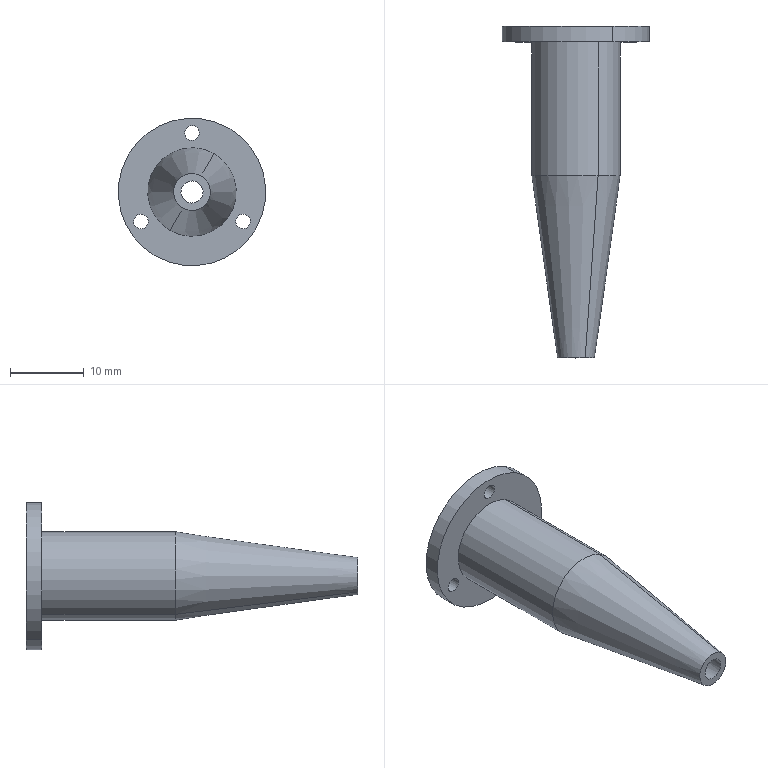Component | SolidWorks | Nozzle2-1 | 1 solid | 21 faces | box 20 x 45 x 20 mm | volume 1658 mm3 | cylinder 12 | cone 6 | plane 3 | commonest cylinder face diameters 2 x6 10 x2 20 x2 12 x2
build123d program:
from build123d import *

# Parameters (mm, degrees)
CUT_EXTRUDE1_REACH = 49.17
SKETCH2_R          = 1


with BuildPart() as part:
    # Sketch1 → Revolve1 (revolve)
    with BuildSketch(Plane.XY, mode=Mode.PRIVATE) as revolve1_sk:
        Polygon((-17.802, 0), (27.198, 0), (27.198, 2.5), (2.473, 6), (-15.659, 6), (-15.659, 10), (-17.802, 10), align=None)
    revolve(revolve1_sk.sketch.rotate(Axis((-17.802, 0, 0), (1, 0, 0)), 90), axis=Axis((-17.802, 0, 0), (1, 0, 0)))

    # Sketch2 → Cut-Extrude1 (cut, up to next)
    with BuildSketch(Plane.ZY.offset(17.802), mode=Mode.PRIVATE) as cut_extrude1_sk1:
        with Locations((0, 8)):
            Circle(SKETCH2_R)
    cut_extrude1_tool1 = extrude(cut_extrude1_sk1.sketch, amount=-CUT_EXTRUDE1_REACH, mode=Mode.PRIVATE) & part.part
    # Sketch2 → Cut-Extrude1 (cut, up to next)
    with BuildSketch(Plane.ZY.offset(17.802), mode=Mode.PRIVATE) as cut_extrude1_sk2:
        with Locations((6.928, -4)):
            Circle(SKETCH2_R)
    cut_extrude1_tool2 = extrude(cut_extrude1_sk2.sketch, amount=-CUT_EXTRUDE1_REACH, mode=Mode.PRIVATE) & part.part
    # Sketch2 → Cut-Extrude1 (cut, up to next)
    with BuildSketch(Plane.ZY.offset(17.802), mode=Mode.PRIVATE) as cut_extrude1_sk3:
        with Locations((-6.928, -4)):
            Circle(SKETCH2_R)
    cut_extrude1_tool3 = extrude(cut_extrude1_sk3.sketch, amount=-CUT_EXTRUDE1_REACH, mode=Mode.PRIVATE) & part.part
    add(cut_extrude1_tool1.solids().sort_by_distance((-17.802, 8, 0))[0], mode=Mode.SUBTRACT)
    add(cut_extrude1_tool2.solids().sort_by_distance((-17.802, -4, 6.928))[0], mode=Mode.SUBTRACT)
    add(cut_extrude1_tool3.solids().sort_by_distance((-17.802, -4, -6.928))[0], mode=Mode.SUBTRACT)

    # Sketch5 → Cut-Revolve1 (revolve, cut)
    with BuildSketch(Plane(origin=(0, 0, 0), x_dir=(1, 0, 0), z_dir=(0, 1, 0)), mode=Mode.PRIVATE) as cut_revolve1_sk:
        Polygon((-17.802, 0), (2.473, 0), (27.198, 0), (27.198, 1.5), (2.473, 5), (-15.659, 5), (-17.802, 6), align=None)
    revolve(cut_revolve1_sk.sketch.rotate(Axis((-17.802, 0, 0), (1, 0, 0)), 180), axis=Axis((-17.802, 0, 0), (1, 0, 0)), mode=Mode.SUBTRACT)


solid = part.part

# Placed as in the assembly
solid = solid.moved(Location((-5.981, -125.796, 160), (90, -90, 0)))
STEP:
#1=COLOUR_RGB('',0.7922,0.8196,0.9333);
#2=FILL_AREA_STYLE_COLOUR('',#1);
#3=FILL_AREA_STYLE('',(#2));
#4=SURFACE_STYLE_FILL_AREA(#3);
#5=SURFACE_SIDE_STYLE('',(#4));
#6=SURFACE_STYLE_USAGE(.BOTH.,#5);
#7=PRESENTATION_STYLE_ASSIGNMENT((#6));
#8=CARTESIAN_POINT('',(-0.3339,-4.336,6.129));
#9=VERTEX_POINT('',#8);
#10=CARTESIAN_POINT('',(-0.137,-4.336,6.47));
#11=VERTEX_POINT('',#10);
#12=CARTESIAN_POINT('',(-0.2355,-4.336,6.299));
#13=DIRECTION('',(-0.,1.,0.));
#14=DIRECTION('',(0.5,0.,0.866));
#15=AXIS2_PLACEMENT_3D('',#12,#13,#14);
#16=CIRCLE('',#15,0.1969);
#17=EDGE_CURVE('',#9,#11,#16,.T.);
#18=ORIENTED_EDGE('',*,*,#17,.F.);
#19=CARTESIAN_POINT('',(-0.3536,-4.252,6.095));
#20=VERTEX_POINT('',#19);
#21=CARTESIAN_POINT('',(-0.3339,-4.336,6.129));
#22=DIRECTION('',(-0.2114,0.9062,-0.3662));
#23=VECTOR('',#22,39.37);
#24=LINE('',#21,#23);
#25=EDGE_CURVE('',#9,#20,#24,.T.);
#26=ORIENTED_EDGE('',*,*,#25,.T.);
#27=CARTESIAN_POINT('',(-0.1174,-4.252,6.504));
#28=VERTEX_POINT('',#27);
#29=CARTESIAN_POINT('',(-0.2355,-4.252,6.299));
#30=DIRECTION('',(-0.,1.,0.));
#31=DIRECTION('',(0.5,0.,0.866));
#32=AXIS2_PLACEMENT_3D('',#29,#30,#31);
#33=CIRCLE('',#32,0.2362);
#34=EDGE_CURVE('',#20,#28,#33,.T.);
#35=ORIENTED_EDGE('',*,*,#34,.T.);
#36=CARTESIAN_POINT('',(-0.137,-4.336,6.47));
#37=DIRECTION('',(0.2114,0.9062,0.3662));
#38=VECTOR('',#37,39.37);
#39=LINE('',#36,#38);
#40=EDGE_CURVE('',#11,#28,#39,.T.);
#41=ORIENTED_EDGE('',*,*,#40,.F.);
#42=EDGE_LOOP('',(#18,#26,#35,#41));
#43=FACE_OUTER_BOUND('',#42,.T.);
#44=CARTESIAN_POINT('',(-0.2355,-4.336,6.299));
#45=DIRECTION('',(-0.,1.,0.));
#46=DIRECTION('',(0.5,0.,0.866));
#47=AXIS2_PLACEMENT_3D('',#44,#45,#46);
#48=CONICAL_SURFACE('',#47,0.1969,0.4366);
#49=ADVANCED_FACE('',(#43),#48,.F.);
#50=CARTESIAN_POINT('',(-0.3339,-5.05,6.129));
#51=VERTEX_POINT('',#50);
#52=CARTESIAN_POINT('',(-0.137,-5.05,6.47));
#53=VERTEX_POINT('',#52);
#54=CARTESIAN_POINT('',(-0.2355,-5.05,6.299));
#55=DIRECTION('',(-0.,1.,0.));
#56=DIRECTION('',(0.5,0.,0.866));
#57=AXIS2_PLACEMENT_3D('',#54,#55,#56);
#58=CIRCLE('',#57,0.1969);
#59=EDGE_CURVE('',#51,#53,#58,.T.);
#60=ORIENTED_EDGE('',*,*,#59,.F.);
#61=CARTESIAN_POINT('',(-0.3339,-4.252,6.129));
#62=DIRECTION('',(-0.,1.,0.));
#63=VECTOR('',#62,39.37);
#64=LINE('',#61,#63);
#65=EDGE_CURVE('',#51,#9,#64,.T.);
#66=ORIENTED_EDGE('',*,*,#65,.T.);
#67=ORIENTED_EDGE('',*,*,#17,.T.);
#68=CARTESIAN_POINT('',(-0.137,-4.252,6.47));
#69=DIRECTION('',(-0.,1.,0.));
#70=VECTOR('',#69,39.37);
#71=LINE('',#68,#70);
#72=EDGE_CURVE('',#53,#11,#71,.T.);
#73=ORIENTED_EDGE('',*,*,#72,.F.);
#74=EDGE_LOOP('',(#60,#66,#67,#73));
#75=FACE_OUTER_BOUND('',#74,.T.);
#76=CARTESIAN_POINT('',(-0.2355,-4.252,6.299));
#77=DIRECTION('',(-0.,1.,0.));
#78=DIRECTION('',(0.5,0.,0.866));
#79=AXIS2_PLACEMENT_3D('',#76,#77,#78);
#80=CYLINDRICAL_SURFACE('',#79,0.1969);
#81=ADVANCED_FACE('',(#75),#80,.F.);
#82=CARTESIAN_POINT('',(-0.265,-6.023,6.248));
#83=VERTEX_POINT('',#82);
#84=CARTESIAN_POINT('',(-0.2059,-6.023,6.35));
#85=VERTEX_POINT('',#84);
#86=CARTESIAN_POINT('',(-0.2355,-6.023,6.299));
#87=DIRECTION('',(-0.,1.,0.));
#88=DIRECTION('',(0.5,0.,0.866));
#89=AXIS2_PLACEMENT_3D('',#86,#87,#88);
#90=CIRCLE('',#89,0.05906);
#91=EDGE_CURVE('',#83,#85,#90,.T.);
#92=ORIENTED_EDGE('',*,*,#91,.F.);
#93=CARTESIAN_POINT('',(-0.265,-6.023,6.248));
#94=DIRECTION('',(-0.07008,0.9901,-0.1214));
#95=VECTOR('',#94,39.37);
#96=LINE('',#93,#95);
#97=EDGE_CURVE('',#83,#51,#96,.T.);
#98=ORIENTED_EDGE('',*,*,#97,.T.);
#99=ORIENTED_EDGE('',*,*,#59,.T.);
#100=CARTESIAN_POINT('',(-0.2059,-6.023,6.35));
#101=DIRECTION('',(0.07008,0.9901,0.1214));
#102=VECTOR('',#101,39.37);
#103=LINE('',#100,#102);
#104=EDGE_CURVE('',#85,#53,#103,.T.);
#105=ORIENTED_EDGE('',*,*,#104,.F.);
#106=EDGE_LOOP('',(#92,#98,#99,#105));
#107=FACE_OUTER_BOUND('',#106,.T.);
#108=CARTESIAN_POINT('',(-0.2355,-6.023,6.299));
#109=DIRECTION('',(-0.,1.,0.));
#110=DIRECTION('',(0.5,0.,0.866));
#111=AXIS2_PLACEMENT_3D('',#108,#109,#110);
#112=CONICAL_SURFACE('',#111,0.05906,0.1406);
#113=ADVANCED_FACE('',(#107),#112,.F.);
#114=CARTESIAN_POINT('',(0.05698,-4.336,6.176));
#115=VERTEX_POINT('',#114);
#116=CARTESIAN_POINT('',(0.01761,-4.336,6.108));
#117=VERTEX_POINT('',#116);
#118=CARTESIAN_POINT('',(0.0373,-4.336,6.142));
#119=DIRECTION('',(0.,-1.,-0.));
#120=DIRECTION('',(0.5,0.,0.866));
#121=AXIS2_PLACEMENT_3D('',#118,#119,#120);
#122=CIRCLE('',#121,0.03937);
#123=EDGE_CURVE('',#115,#117,#122,.T.);
#124=ORIENTED_EDGE('',*,*,#123,.T.);
#125=CARTESIAN_POINT('',(0.01761,-4.252,6.108));
#126=VERTEX_POINT('',#125);
#127=CARTESIAN_POINT('',(0.01761,-6.023,6.108));
#128=DIRECTION('',(-0.,1.,0.));
#129=VECTOR('',#128,39.37);
#130=LINE('',#127,#129);
#131=EDGE_CURVE('',#117,#126,#130,.T.);
#132=ORIENTED_EDGE('',*,*,#131,.T.);
#133=CARTESIAN_POINT('',(0.05698,-4.252,6.176));
#134=VERTEX_POINT('',#133);
#135=CARTESIAN_POINT('',(0.0373,-4.252,6.142));
#136=DIRECTION('',(-0.,1.,0.));
#137=DIRECTION('',(0.5,0.,0.866));
#138=AXIS2_PLACEMENT_3D('',#135,#136,#137);
#139=CIRCLE('',#138,0.03937);
#140=EDGE_CURVE('',#126,#134,#139,.T.);
#141=ORIENTED_EDGE('',*,*,#140,.T.);
#142=CARTESIAN_POINT('',(0.05698,-6.023,6.176));
#143=DIRECTION('',(-0.,1.,0.));
#144=VECTOR('',#143,39.37);
#145=LINE('',#142,#144);
#146=EDGE_CURVE('',#115,#134,#145,.T.);
#147=ORIENTED_EDGE('',*,*,#146,.F.);
#148=EDGE_LOOP('',(#124,#132,#141,#147));
#149=FACE_OUTER_BOUND('',#148,.T.);
#150=CARTESIAN_POINT('',(0.0373,-6.023,6.142));
#151=DIRECTION('',(-0.,1.,0.));
#152=DIRECTION('',(0.5,0.,0.866));
#153=AXIS2_PLACEMENT_3D('',#150,#151,#152);
#154=CYLINDRICAL_SURFACE('',#153,0.03937);
#155=ADVANCED_FACE('',(#149),#154,.F.);
#156=CARTESIAN_POINT('',(-0.2158,-4.336,6.648));
#157=VERTEX_POINT('',#156);
#158=CARTESIAN_POINT('',(-0.2552,-4.336,6.58));
#159=VERTEX_POINT('',#158);
#160=CARTESIAN_POINT('',(-0.2355,-4.336,6.614));
#161=DIRECTION('',(0.,-1.,-0.));
#162=DIRECTION('',(0.5,0.,0.866));
#163=AXIS2_PLACEMENT_3D('',#160,#161,#162);
#164=CIRCLE('',#163,0.03937);
#165=EDGE_CURVE('',#157,#159,#164,.T.);
#166=ORIENTED_EDGE('',*,*,#165,.T.);
#167=CARTESIAN_POINT('',(-0.2552,-4.252,6.58));
#168=VERTEX_POINT('',#167);
#169=CARTESIAN_POINT('',(-0.2552,-6.023,6.58));
#170=DIRECTION('',(-0.,1.,0.));
#171=VECTOR('',#170,39.37);
#172=LINE('',#169,#171);
#173=EDGE_CURVE('',#159,#168,#172,.T.);
#174=ORIENTED_EDGE('',*,*,#173,.T.);
#175=CARTESIAN_POINT('',(-0.2158,-4.252,6.648));
#176=VERTEX_POINT('',#175);
#177=CARTESIAN_POINT('',(-0.2355,-4.252,6.614));
#178=DIRECTION('',(-0.,1.,0.));
#179=DIRECTION('',(0.5,0.,0.866));
#180=AXIS2_PLACEMENT_3D('',#177,#178,#179);
#181=CIRCLE('',#180,0.03937);
#182=EDGE_CURVE('',#168,#176,#181,.T.);
#183=ORIENTED_EDGE('',*,*,#182,.T.);
#184=CARTESIAN_POINT('',(-0.2158,-6.023,6.648));
#185=DIRECTION('',(-0.,1.,0.));
#186=VECTOR('',#185,39.37);
#187=LINE('',#184,#186);
#188=EDGE_CURVE('',#157,#176,#187,.T.);
#189=ORIENTED_EDGE('',*,*,#188,.F.);
#190=EDGE_LOOP('',(#166,#174,#183,#189));
#191=FACE_OUTER_BOUND('',#190,.T.);
#192=CARTESIAN_POINT('',(-0.2355,-6.023,6.614));
#193=DIRECTION('',(-0.,1.,0.));
#194=DIRECTION('',(0.5,0.,0.866));
#195=AXIS2_PLACEMENT_3D('',#192,#193,#194);
#196=CYLINDRICAL_SURFACE('',#195,0.03937);
#197=ADVANCED_FACE('',(#191),#196,.F.);
#198=CARTESIAN_POINT('',(-0.4885,-4.336,6.176));
#199=VERTEX_POINT('',#198);
#200=CARTESIAN_POINT('',(-0.5279,-4.336,6.108));
#201=VERTEX_POINT('',#200);
#202=CARTESIAN_POINT('',(-0.5082,-4.336,6.142));
#203=DIRECTION('',(0.,-1.,-0.));
#204=DIRECTION('',(0.5,0.,0.866));
#205=AXIS2_PLACEMENT_3D('',#202,#203,#204);
#206=CIRCLE('',#205,0.03937);
#207=EDGE_CURVE('',#199,#201,#206,.T.);
#208=ORIENTED_EDGE('',*,*,#207,.T.);
#209=CARTESIAN_POINT('',(-0.5279,-4.252,6.108));
#210=VERTEX_POINT('',#209);
#211=CARTESIAN_POINT('',(-0.5279,-6.023,6.108));
#212=DIRECTION('',(-0.,1.,0.));
#213=VECTOR('',#212,39.37);
#214=LINE('',#211,#213);
#215=EDGE_CURVE('',#201,#210,#214,.T.);
#216=ORIENTED_EDGE('',*,*,#215,.T.);
#217=CARTESIAN_POINT('',(-0.4885,-4.252,6.176));
#218=VERTEX_POINT('',#217);
#219=CARTESIAN_POINT('',(-0.5082,-4.252,6.142));
#220=DIRECTION('',(-0.,1.,0.));
#221=DIRECTION('',(0.5,0.,0.866));
#222=AXIS2_PLACEMENT_3D('',#219,#220,#221);
#223=CIRCLE('',#222,0.03937);
#224=EDGE_CURVE('',#210,#218,#223,.T.);
#225=ORIENTED_EDGE('',*,*,#224,.T.);
#226=CARTESIAN_POINT('',(-0.4885,-6.023,6.176));
#227=DIRECTION('',(-0.,1.,0.));
#228=VECTOR('',#227,39.37);
#229=LINE('',#226,#228);
#230=EDGE_CURVE('',#199,#218,#229,.T.);
#231=ORIENTED_EDGE('',*,*,#230,.F.);
#232=EDGE_LOOP('',(#208,#216,#225,#231));
#233=FACE_OUTER_BOUND('',#232,.T.);
#234=CARTESIAN_POINT('',(-0.5082,-6.023,6.142));
#235=DIRECTION('',(-0.,1.,0.));
#236=DIRECTION('',(0.5,0.,0.866));
#237=AXIS2_PLACEMENT_3D('',#234,#235,#236);
#238=CYLINDRICAL_SURFACE('',#237,0.03937);
#239=ADVANCED_FACE('',(#233),#238,.F.);
#240=CARTESIAN_POINT('',(-0.03862,-4.336,6.64));
#241=VERTEX_POINT('',#240);
#242=CARTESIAN_POINT('',(-0.4323,-4.336,5.958));
#243=VERTEX_POINT('',#242);
#244=CARTESIAN_POINT('',(-0.2355,-4.336,6.299));
#245=DIRECTION('',(-0.,1.,0.));
#246=DIRECTION('',(0.5,0.,0.866));
#247=AXIS2_PLACEMENT_3D('',#244,#245,#246);
#248=CIRCLE('',#247,0.3937);
#249=EDGE_CURVE('',#241,#243,#248,.T.);
#250=ORIENTED_EDGE('',*,*,#249,.T.);
#251=CARTESIAN_POINT('',(-0.4323,-4.252,5.958));
#252=VERTEX_POINT('',#251);
#253=CARTESIAN_POINT('',(-0.4323,-4.252,5.958));
#254=DIRECTION('',(-0.,1.,0.));
#255=VECTOR('',#254,39.37);
#256=LINE('',#253,#255);
#257=EDGE_CURVE('',#243,#252,#256,.T.);
#258=ORIENTED_EDGE('',*,*,#257,.T.);
#259=CARTESIAN_POINT('',(-0.03862,-4.252,6.64));
#260=VERTEX_POINT('',#259);
#261=CARTESIAN_POINT('',(-0.2355,-4.252,6.299));
#262=DIRECTION('',(-0.,1.,0.));
#263=DIRECTION('',(0.5,0.,0.866));
#264=AXIS2_PLACEMENT_3D('',#261,#262,#263);
#265=CIRCLE('',#264,0.3937);
#266=EDGE_CURVE('',#260,#252,#265,.T.);
#267=ORIENTED_EDGE('',*,*,#266,.F.);
#268=CARTESIAN_POINT('',(-0.03862,-4.252,6.64));
#269=DIRECTION('',(-0.,1.,0.));
#270=VECTOR('',#269,39.37);
#271=LINE('',#268,#270);
#272=EDGE_CURVE('',#241,#260,#271,.T.);
#273=ORIENTED_EDGE('',*,*,#272,.F.);
#274=EDGE_LOOP('',(#250,#258,#267,#273));
#275=FACE_OUTER_BOUND('',#274,.T.);
#276=CARTESIAN_POINT('',(-0.2355,-4.252,6.299));
#277=DIRECTION('',(-0.,1.,0.));
#278=DIRECTION('',(0.5,0.,0.866));
#279=AXIS2_PLACEMENT_3D('',#276,#277,#278);
#280=CYLINDRICAL_SURFACE('',#279,0.3937);
#281=ADVANCED_FACE('',(#275),#280,.T.);
#282=CARTESIAN_POINT('',(-0.1174,-5.05,6.504));
#283=VERTEX_POINT('',#282);
#284=CARTESIAN_POINT('',(-0.3536,-5.05,6.095));
#285=VERTEX_POINT('',#284);
#286=CARTESIAN_POINT('',(-0.2355,-5.05,6.299));
#287=DIRECTION('',(-0.,1.,0.));
#288=DIRECTION('',(0.5,0.,0.866));
#289=AXIS2_PLACEMENT_3D('',#286,#287,#288);
#290=CIRCLE('',#289,0.2362);
#291=EDGE_CURVE('',#283,#285,#290,.T.);
#292=ORIENTED_EDGE('',*,*,#291,.T.);
#293=CARTESIAN_POINT('',(-0.3536,-4.336,6.095));
#294=VERTEX_POINT('',#293);
#295=CARTESIAN_POINT('',(-0.3536,-4.252,6.095));
#296=DIRECTION('',(-0.,1.,0.));
#297=VECTOR('',#296,39.37);
#298=LINE('',#295,#297);
#299=EDGE_CURVE('',#285,#294,#298,.T.);
#300=ORIENTED_EDGE('',*,*,#299,.T.);
#301=CARTESIAN_POINT('',(-0.1174,-4.336,6.504));
#302=VERTEX_POINT('',#301);
#303=CARTESIAN_POINT('',(-0.2355,-4.336,6.299));
#304=DIRECTION('',(-0.,1.,0.));
#305=DIRECTION('',(0.5,0.,0.866));
#306=AXIS2_PLACEMENT_3D('',#303,#304,#305);
#307=CIRCLE('',#306,0.2362);
#308=EDGE_CURVE('',#302,#294,#307,.T.);
#309=ORIENTED_EDGE('',*,*,#308,.F.);
#310=CARTESIAN_POINT('',(-0.1174,-4.252,6.504));
#311=DIRECTION('',(-0.,1.,0.));
#312=VECTOR('',#311,39.37);
#313=LINE('',#310,#312);
#314=EDGE_CURVE('',#283,#302,#313,.T.);
#315=ORIENTED_EDGE('',*,*,#314,.F.);
#316=EDGE_LOOP('',(#292,#300,#309,#315));
#317=FACE_OUTER_BOUND('',#316,.T.);
#318=CARTESIAN_POINT('',(-0.2355,-4.252,6.299));
#319=DIRECTION('',(-0.,1.,0.));
#320=DIRECTION('',(0.5,0.,0.866));
#321=AXIS2_PLACEMENT_3D('',#318,#319,#320);
#322=CYLINDRICAL_SURFACE('',#321,0.2362);
#323=ADVANCED_FACE('',(#317),#322,.T.);
#324=CARTESIAN_POINT('',(-0.1863,-6.023,6.384));
#325=VERTEX_POINT('',#324);
#326=CARTESIAN_POINT('',(-0.2847,-6.023,6.214));
#327=VERTEX_POINT('',#326);
#328=CARTESIAN_POINT('',(-0.2355,-6.023,6.299));
#329=DIRECTION('',(-0.,1.,0.));
#330=DIRECTION('',(0.5,0.,0.866));
#331=AXIS2_PLACEMENT_3D('',#328,#329,#330);
#332=CIRCLE('',#331,0.09843);
#333=EDGE_CURVE('',#325,#327,#332,.T.);
#334=ORIENTED_EDGE('',*,*,#333,.T.);
#335=CARTESIAN_POINT('',(-0.2847,-6.023,6.214));
#336=DIRECTION('',(-0.07008,0.9901,-0.1214));
#337=VECTOR('',#336,39.37);
#338=LINE('',#335,#337);
#339=EDGE_CURVE('',#327,#285,#338,.T.);
#340=ORIENTED_EDGE('',*,*,#339,.T.);
#341=ORIENTED_EDGE('',*,*,#291,.F.);
#342=CARTESIAN_POINT('',(-0.1863,-6.023,6.384));
#343=DIRECTION('',(0.07008,0.9901,0.1214));
#344=VECTOR('',#343,39.37);
#345=LINE('',#342,#344);
#346=EDGE_CURVE('',#325,#283,#345,.T.);
#347=ORIENTED_EDGE('',*,*,#346,.F.);
#348=EDGE_LOOP('',(#334,#340,#341,#347));
#349=FACE_OUTER_BOUND('',#348,.T.);
#350=CARTESIAN_POINT('',(-0.2355,-6.023,6.299));
#351=DIRECTION('',(-0.,1.,0.));
#352=DIRECTION('',(0.5,0.,0.866));
#353=AXIS2_PLACEMENT_3D('',#350,#351,#352);
#354=CONICAL_SURFACE('',#353,0.09843,0.1406);
#355=ADVANCED_FACE('',(#349),#354,.T.);
#356=CARTESIAN_POINT('',(-0.2355,-4.252,6.299));
#357=DIRECTION('',(-0.,1.,0.));
#358=DIRECTION('',(0.5,0.,0.866));
#359=AXIS2_PLACEMENT_3D('',#356,#357,#358);
#360=CIRCLE('',#359,0.2362);
#361=EDGE_CURVE('',#28,#20,#360,.T.);
#362=ORIENTED_EDGE('',*,*,#361,.F.);
#363=ORIENTED_EDGE('',*,*,#34,.F.);
#364=EDGE_LOOP('',(#362,#363));
#365=FACE_BOUND('',#364,.T.);
#366=CARTESIAN_POINT('',(0.0373,-4.252,6.142));
#367=DIRECTION('',(-0.,1.,0.));
#368=DIRECTION('',(0.5,0.,0.866));
#369=AXIS2_PLACEMENT_3D('',#366,#367,#368);
#370=CIRCLE('',#369,0.03937);
#371=EDGE_CURVE('',#134,#126,#370,.T.);
#372=ORIENTED_EDGE('',*,*,#371,.F.);
#373=ORIENTED_EDGE('',*,*,#140,.F.);
#374=EDGE_LOOP('',(#372,#373));
#375=FACE_BOUND('',#374,.T.);
#376=CARTESIAN_POINT('',(-0.2355,-4.252,6.614));
#377=DIRECTION('',(-0.,1.,0.));
#378=DIRECTION('',(0.5,0.,0.866));
#379=AXIS2_PLACEMENT_3D('',#376,#377,#378);
#380=CIRCLE('',#379,0.03937);
#381=EDGE_CURVE('',#176,#168,#380,.T.);
#382=ORIENTED_EDGE('',*,*,#381,.F.);
#383=ORIENTED_EDGE('',*,*,#182,.F.);
#384=EDGE_LOOP('',(#382,#383));
#385=FACE_BOUND('',#384,.T.);
#386=CARTESIAN_POINT('',(-0.5082,-4.252,6.142));
#387=DIRECTION('',(-0.,1.,0.));
#388=DIRECTION('',(0.5,0.,0.866));
#389=AXIS2_PLACEMENT_3D('',#386,#387,#388);
#390=CIRCLE('',#389,0.03937);
#391=EDGE_CURVE('',#218,#210,#390,.T.);
#392=ORIENTED_EDGE('',*,*,#391,.F.);
#393=ORIENTED_EDGE('',*,*,#224,.F.);
#394=EDGE_LOOP('',(#392,#393));
#395=FACE_BOUND('',#394,.T.);
#396=ORIENTED_EDGE('',*,*,#266,.T.);
#397=CARTESIAN_POINT('',(-0.2355,-4.252,6.299));
#398=DIRECTION('',(-0.,1.,0.));
#399=DIRECTION('',(0.5,0.,0.866));
#400=AXIS2_PLACEMENT_3D('',#397,#398,#399);
#401=CIRCLE('',#400,0.3937);
#402=EDGE_CURVE('',#252,#260,#401,.T.);
#403=ORIENTED_EDGE('',*,*,#402,.T.);
#404=EDGE_LOOP('',(#396,#403));
#405=FACE_OUTER_BOUND('',#404,.T.);
#406=CARTESIAN_POINT('',(0.1055,-4.252,6.102));
#407=DIRECTION('',(0.,-1.,-0.));
#408=DIRECTION('',(-0.5,0.,-0.866));
#409=AXIS2_PLACEMENT_3D('',#406,#407,#408);
#410=PLANE('',#409);
#411=ADVANCED_FACE('',(#365,#375,#385,#395,#405),#410,.F.);
#412=CARTESIAN_POINT('',(-0.2355,-6.023,6.299));
#413=DIRECTION('',(-0.,1.,0.));
#414=DIRECTION('',(0.5,0.,0.866));
#415=AXIS2_PLACEMENT_3D('',#412,#413,#414);
#416=CIRCLE('',#415,0.05906);
#417=EDGE_CURVE('',#85,#83,#416,.T.);
#418=ORIENTED_EDGE('',*,*,#417,.T.);
#419=ORIENTED_EDGE('',*,*,#91,.T.);
#420=EDGE_LOOP('',(#418,#419));
#421=FACE_BOUND('',#420,.T.);
#422=ORIENTED_EDGE('',*,*,#333,.F.);
#423=CARTESIAN_POINT('',(-0.2355,-6.023,6.299));
#424=DIRECTION('',(-0.,1.,0.));
#425=DIRECTION('',(0.5,0.,0.866));
#426=AXIS2_PLACEMENT_3D('',#423,#424,#425);
#427=CIRCLE('',#426,0.09843);
#428=EDGE_CURVE('',#327,#325,#427,.T.);
#429=ORIENTED_EDGE('',*,*,#428,.F.);
#430=EDGE_LOOP('',(#422,#429));
#431=FACE_OUTER_BOUND('',#430,.T.);
#432=CARTESIAN_POINT('',(-0.2355,-6.023,6.299));
#433=DIRECTION('',(-0.,1.,0.));
#434=DIRECTION('',(0.5,-0.,0.866));
#435=AXIS2_PLACEMENT_3D('',#432,#433,#434);
#436=PLANE('',#435);
#437=ADVANCED_FACE('',(#421,#431),#436,.F.);
#438=ORIENTED_EDGE('',*,*,#339,.F.);
#439=ORIENTED_EDGE('',*,*,#428,.T.);
#440=ORIENTED_EDGE('',*,*,#346,.T.);
#441=CARTESIAN_POINT('',(-0.2355,-5.05,6.299));
#442=DIRECTION('',(-0.,1.,0.));
#443=DIRECTION('',(0.5,0.,0.866));
#444=AXIS2_PLACEMENT_3D('',#441,#442,#443);
#445=CIRCLE('',#444,0.2362);
#446=EDGE_CURVE('',#285,#283,#445,.T.);
#447=ORIENTED_EDGE('',*,*,#446,.F.);
#448=EDGE_LOOP('',(#438,#439,#440,#447));
#449=FACE_OUTER_BOUND('',#448,.T.);
#450=CARTESIAN_POINT('',(-0.2355,-6.023,6.299));
#451=DIRECTION('',(-0.,1.,0.));
#452=DIRECTION('',(0.5,0.,0.866));
#453=AXIS2_PLACEMENT_3D('',#450,#451,#452);
#454=CONICAL_SURFACE('',#453,0.09843,0.1406);
#455=ADVANCED_FACE('',(#449),#454,.T.);
#456=ORIENTED_EDGE('',*,*,#299,.F.);
#457=ORIENTED_EDGE('',*,*,#446,.T.);
#458=ORIENTED_EDGE('',*,*,#314,.T.);
#459=CARTESIAN_POINT('',(-0.2355,-4.336,6.299));
#460=DIRECTION('',(-0.,1.,0.));
#461=DIRECTION('',(0.5,0.,0.866));
#462=AXIS2_PLACEMENT_3D('',#459,#460,#461);
#463=CIRCLE('',#462,0.2362);
#464=EDGE_CURVE('',#294,#302,#463,.T.);
#465=ORIENTED_EDGE('',*,*,#464,.F.);
#466=EDGE_LOOP('',(#456,#457,#458,#465));
#467=FACE_OUTER_BOUND('',#466,.T.);
#468=CARTESIAN_POINT('',(-0.2355,-4.252,6.299));
#469=DIRECTION('',(-0.,1.,0.));
#470=DIRECTION('',(0.5,0.,0.866));
#471=AXIS2_PLACEMENT_3D('',#468,#469,#470);
#472=CYLINDRICAL_SURFACE('',#471,0.2362);
#473=ADVANCED_FACE('',(#467),#472,.T.);
#474=ORIENTED_EDGE('',*,*,#123,.F.);
#475=CARTESIAN_POINT('',(0.0373,-4.336,6.142));
#476=DIRECTION('',(0.,-1.,-0.));
#477=DIRECTION('',(0.5,0.,0.866));
#478=AXIS2_PLACEMENT_3D('',#475,#476,#477);
#479=CIRCLE('',#478,0.03937);
#480=EDGE_CURVE('',#117,#115,#479,.T.);
#481=ORIENTED_EDGE('',*,*,#480,.F.);
#482=EDGE_LOOP('',(#474,#481));
#483=FACE_BOUND('',#482,.T.);
#484=ORIENTED_EDGE('',*,*,#165,.F.);
#485=CARTESIAN_POINT('',(-0.2355,-4.336,6.614));
#486=DIRECTION('',(0.,-1.,-0.));
#487=DIRECTION('',(0.5,0.,0.866));
#488=AXIS2_PLACEMENT_3D('',#485,#486,#487);
#489=CIRCLE('',#488,0.03937);
#490=EDGE_CURVE('',#159,#157,#489,.T.);
#491=ORIENTED_EDGE('',*,*,#490,.F.);
#492=EDGE_LOOP('',(#484,#491));
#493=FACE_BOUND('',#492,.T.);
#494=ORIENTED_EDGE('',*,*,#207,.F.);
#495=CARTESIAN_POINT('',(-0.5082,-4.336,6.142));
#496=DIRECTION('',(0.,-1.,-0.));
#497=DIRECTION('',(0.5,0.,0.866));
#498=AXIS2_PLACEMENT_3D('',#495,#496,#497);
#499=CIRCLE('',#498,0.03937);
#500=EDGE_CURVE('',#201,#199,#499,.T.);
#501=ORIENTED_EDGE('',*,*,#500,.F.);
#502=EDGE_LOOP('',(#494,#501));
#503=FACE_BOUND('',#502,.T.);
#504=ORIENTED_EDGE('',*,*,#249,.F.);
#505=CARTESIAN_POINT('',(-0.2355,-4.336,6.299));
#506=DIRECTION('',(-0.,1.,0.));
#507=DIRECTION('',(0.5,0.,0.866));
#508=AXIS2_PLACEMENT_3D('',#505,#506,#507);
#509=CIRCLE('',#508,0.3937);
#510=EDGE_CURVE('',#243,#241,#509,.T.);
#511=ORIENTED_EDGE('',*,*,#510,.F.);
#512=EDGE_LOOP('',(#504,#511));
#513=FACE_OUTER_BOUND('',#512,.T.);
#514=ORIENTED_EDGE('',*,*,#308,.T.);
#515=ORIENTED_EDGE('',*,*,#464,.T.);
#516=EDGE_LOOP('',(#514,#515));
#517=FACE_BOUND('',#516,.T.);
#518=CARTESIAN_POINT('',(-0.0309,-4.336,6.181));
#519=DIRECTION('',(-0.,1.,0.));
#520=DIRECTION('',(0.5,-0.,0.866));
#521=AXIS2_PLACEMENT_3D('',#518,#519,#520);
#522=PLANE('',#521);
#523=ADVANCED_FACE('',(#483,#493,#503,#513,#517),#522,.F.);
#524=ORIENTED_EDGE('',*,*,#257,.F.);
#525=ORIENTED_EDGE('',*,*,#510,.T.);
#526=ORIENTED_EDGE('',*,*,#272,.T.);
#527=ORIENTED_EDGE('',*,*,#402,.F.);
#528=EDGE_LOOP('',(#524,#525,#526,#527));
#529=FACE_OUTER_BOUND('',#528,.T.);
#530=CARTESIAN_POINT('',(-0.2355,-4.252,6.299));
#531=DIRECTION('',(-0.,1.,0.));
#532=DIRECTION('',(0.5,0.,0.866));
#533=AXIS2_PLACEMENT_3D('',#530,#531,#532);
#534=CYLINDRICAL_SURFACE('',#533,0.3937);
#535=ADVANCED_FACE('',(#529),#534,.T.);
#536=ORIENTED_EDGE('',*,*,#215,.F.);
#537=ORIENTED_EDGE('',*,*,#500,.T.);
#538=ORIENTED_EDGE('',*,*,#230,.T.);
#539=ORIENTED_EDGE('',*,*,#391,.T.);
#540=EDGE_LOOP('',(#536,#537,#538,#539));
#541=FACE_OUTER_BOUND('',#540,.T.);
#542=CARTESIAN_POINT('',(-0.5082,-6.023,6.142));
#543=DIRECTION('',(-0.,1.,0.));
#544=DIRECTION('',(0.5,0.,0.866));
#545=AXIS2_PLACEMENT_3D('',#542,#543,#544);
#546=CYLINDRICAL_SURFACE('',#545,0.03937);
#547=ADVANCED_FACE('',(#541),#546,.F.);
#548=ORIENTED_EDGE('',*,*,#173,.F.);
#549=ORIENTED_EDGE('',*,*,#490,.T.);
#550=ORIENTED_EDGE('',*,*,#188,.T.);
#551=ORIENTED_EDGE('',*,*,#381,.T.);
#552=EDGE_LOOP('',(#548,#549,#550,#551));
#553=FACE_OUTER_BOUND('',#552,.T.);
#554=CARTESIAN_POINT('',(-0.2355,-6.023,6.614));
#555=DIRECTION('',(-0.,1.,0.));
#556=DIRECTION('',(0.5,0.,0.866));
#557=AXIS2_PLACEMENT_3D('',#554,#555,#556);
#558=CYLINDRICAL_SURFACE('',#557,0.03937);
#559=ADVANCED_FACE('',(#553),#558,.F.);
#560=ORIENTED_EDGE('',*,*,#131,.F.);
#561=ORIENTED_EDGE('',*,*,#480,.T.);
#562=ORIENTED_EDGE('',*,*,#146,.T.);
#563=ORIENTED_EDGE('',*,*,#371,.T.);
#564=EDGE_LOOP('',(#560,#561,#562,#563));
#565=FACE_OUTER_BOUND('',#564,.T.);
#566=CARTESIAN_POINT('',(0.0373,-6.023,6.142));
#567=DIRECTION('',(-0.,1.,0.));
#568=DIRECTION('',(0.5,0.,0.866));
#569=AXIS2_PLACEMENT_3D('',#566,#567,#568);
#570=CYLINDRICAL_SURFACE('',#569,0.03937);
#571=ADVANCED_FACE('',(#565),#570,.F.);
#572=ORIENTED_EDGE('',*,*,#97,.F.);
#573=ORIENTED_EDGE('',*,*,#417,.F.);
#574=ORIENTED_EDGE('',*,*,#104,.T.);
#575=CARTESIAN_POINT('',(-0.2355,-5.05,6.299));
#576=DIRECTION('',(-0.,1.,0.));
#577=DIRECTION('',(0.5,0.,0.866));
#578=AXIS2_PLACEMENT_3D('',#575,#576,#577);
#579=CIRCLE('',#578,0.1969);
#580=EDGE_CURVE('',#53,#51,#579,.T.);
#581=ORIENTED_EDGE('',*,*,#580,.T.);
#582=EDGE_LOOP('',(#572,#573,#574,#581));
#583=FACE_OUTER_BOUND('',#582,.T.);
#584=CARTESIAN_POINT('',(-0.2355,-6.023,6.299));
#585=DIRECTION('',(-0.,1.,0.));
#586=DIRECTION('',(0.5,0.,0.866));
#587=AXIS2_PLACEMENT_3D('',#584,#585,#586);
#588=CONICAL_SURFACE('',#587,0.05906,0.1406);
#589=ADVANCED_FACE('',(#583),#588,.F.);
#590=ORIENTED_EDGE('',*,*,#65,.F.);
#591=ORIENTED_EDGE('',*,*,#580,.F.);
#592=ORIENTED_EDGE('',*,*,#72,.T.);
#593=CARTESIAN_POINT('',(-0.2355,-4.336,6.299));
#594=DIRECTION('',(-0.,1.,0.));
#595=DIRECTION('',(0.5,0.,0.866));
#596=AXIS2_PLACEMENT_3D('',#593,#594,#595);
#597=CIRCLE('',#596,0.1969);
#598=EDGE_CURVE('',#11,#9,#597,.T.);
#599=ORIENTED_EDGE('',*,*,#598,.T.);
#600=EDGE_LOOP('',(#590,#591,#592,#599));
#601=FACE_OUTER_BOUND('',#600,.T.);
#602=CARTESIAN_POINT('',(-0.2355,-4.252,6.299));
#603=DIRECTION('',(-0.,1.,0.));
#604=DIRECTION('',(0.5,0.,0.866));
#605=AXIS2_PLACEMENT_3D('',#602,#603,#604);
#606=CYLINDRICAL_SURFACE('',#605,0.1969);
#607=ADVANCED_FACE('',(#601),#606,.F.);
#608=ORIENTED_EDGE('',*,*,#25,.F.);
#609=ORIENTED_EDGE('',*,*,#598,.F.);
#610=ORIENTED_EDGE('',*,*,#40,.T.);
#611=ORIENTED_EDGE('',*,*,#361,.T.);
#612=EDGE_LOOP('',(#608,#609,#610,#611));
#613=FACE_OUTER_BOUND('',#612,.T.);
#614=CARTESIAN_POINT('',(-0.2355,-4.336,6.299));
#615=DIRECTION('',(-0.,1.,0.));
#616=DIRECTION('',(0.5,0.,0.866));
#617=AXIS2_PLACEMENT_3D('',#614,#615,#616);
#618=CONICAL_SURFACE('',#617,0.1969,0.4366);
#619=ADVANCED_FACE('',(#613),#618,.F.);
#620=CLOSED_SHELL('',(#49,#81,#113,#155,#197,#239,#281,#323,#355,#411,#437,#455,#473,#523,#535,#547,#559,#571,#589,#607,#619));
#621=MANIFOLD_SOLID_BREP('',#620);
#622=STYLED_ITEM('',(#7),#621);
#623=PRESENTATION_LAYER_ASSIGNMENT('','',(#622));
#624=CARTESIAN_POINT('',(0.,0.,0.));
#625=DIRECTION('',(0.,0.,1.));
#626=DIRECTION('',(1.,0.,0.));
#627=AXIS2_PLACEMENT_3D('',#624,#625,#626);
#628=(LENGTH_UNIT()NAMED_UNIT(*)SI_UNIT($,.METRE.));
#629=LENGTH_MEASURE_WITH_UNIT(LENGTH_MEASURE(0.0254),#628);
#630=DIMENSIONAL_EXPONENTS(1.,0.,0.,0.,0.,0.,0.);
#631=(CONVERSION_BASED_UNIT('',#629)LENGTH_UNIT()NAMED_UNIT(#630));
#632=UNCERTAINTY_MEASURE_WITH_UNIT(LENGTH_MEASURE(0.00001),#631,'','');
#633=(NAMED_UNIT(*)PLANE_ANGLE_UNIT()SI_UNIT($,.RADIAN.));
#634=(NAMED_UNIT(*)SI_UNIT($,.STERADIAN.)SOLID_ANGLE_UNIT());
#635=(GEOMETRIC_REPRESENTATION_CONTEXT(3)GLOBAL_UNCERTAINTY_ASSIGNED_CONTEXT((#632))GLOBAL_UNIT_ASSIGNED_CONTEXT((#631,#633,#634))REPRESENTATION_CONTEXT('',''));
#636=ADVANCED_BREP_SHAPE_REPRESENTATION('',(#621,#627),#635);
#637=(LENGTH_UNIT()NAMED_UNIT(*)SI_UNIT($,.METRE.));
#638=LENGTH_MEASURE_WITH_UNIT(LENGTH_MEASURE(0.0254),#637);
#639=DIMENSIONAL_EXPONENTS(1.,0.,0.,0.,0.,0.,0.);
#640=(CONVERSION_BASED_UNIT('',#638)LENGTH_UNIT()NAMED_UNIT(#639));
#641=UNCERTAINTY_MEASURE_WITH_UNIT(LENGTH_MEASURE(0.00001),#640,'','');
#642=(NAMED_UNIT(*)PLANE_ANGLE_UNIT()SI_UNIT($,.RADIAN.));
#643=(NAMED_UNIT(*)SI_UNIT($,.STERADIAN.)SOLID_ANGLE_UNIT());
#644=(GEOMETRIC_REPRESENTATION_CONTEXT(3)GLOBAL_UNCERTAINTY_ASSIGNED_CONTEXT((#641))GLOBAL_UNIT_ASSIGNED_CONTEXT((#640,#642,#643))REPRESENTATION_CONTEXT('',''));
#645=MECHANICAL_DESIGN_GEOMETRIC_PRESENTATION_REPRESENTATION('',(#622),#644);